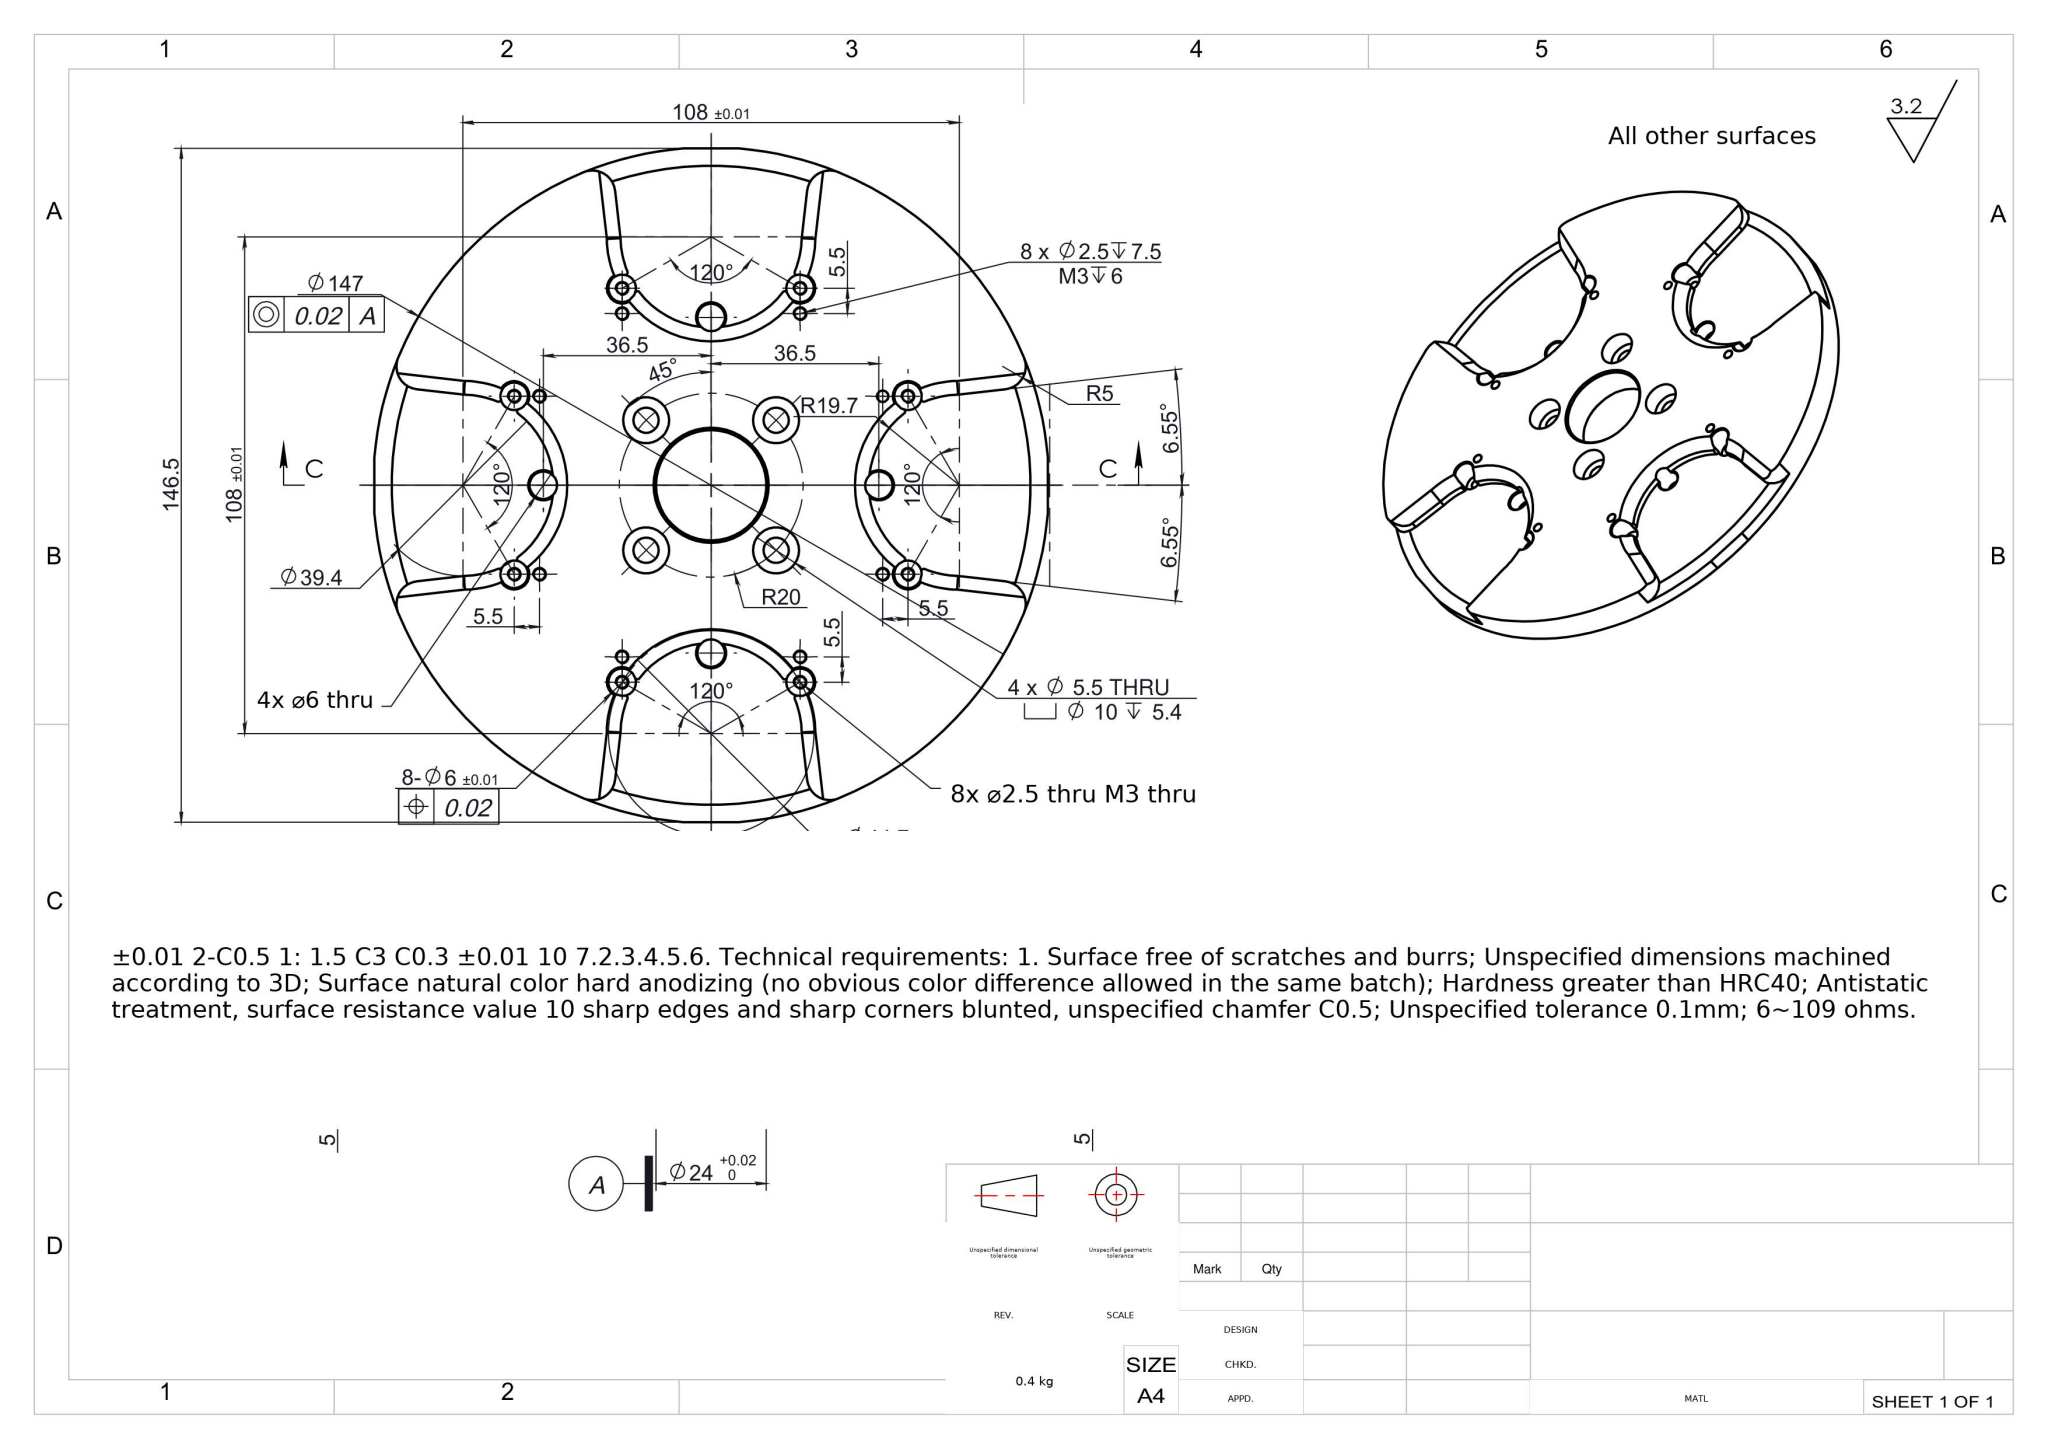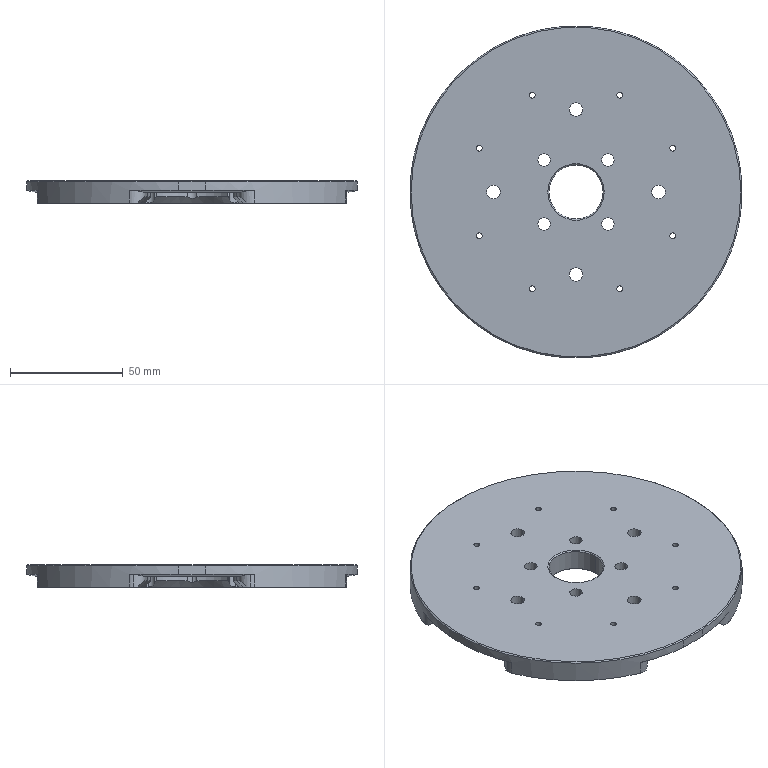Part | SolidWorks | mm | 1 solid | 225 faces | box 146.5 x 146.5 x 10 mm | volume 130750 mm3 | cylinder 126 | cone 61 | plane 38 | commonest cylinder face diameters 2.5 x32 6 x24 1 x22 10 x18 39.4 x16 5.5 x8 147 x4 24 x2